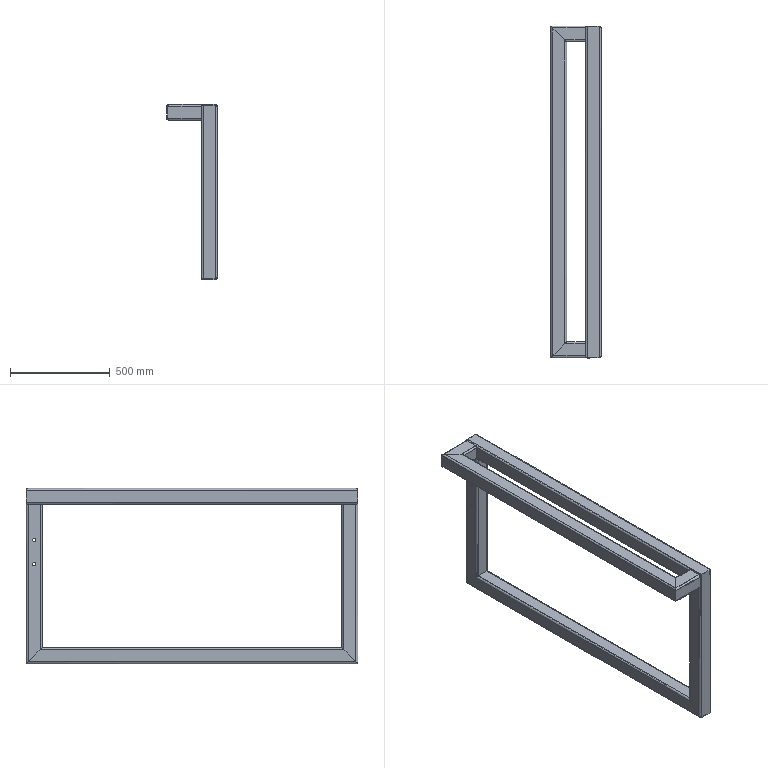Component | SolidWorks | 6.1Frame-1 | 7 solids | 134 faces | volume 9500027 mm3 | plane 70 | cylinder 64 | commonest cylinder face diameters 20 x28 10 x28 15.5 x8